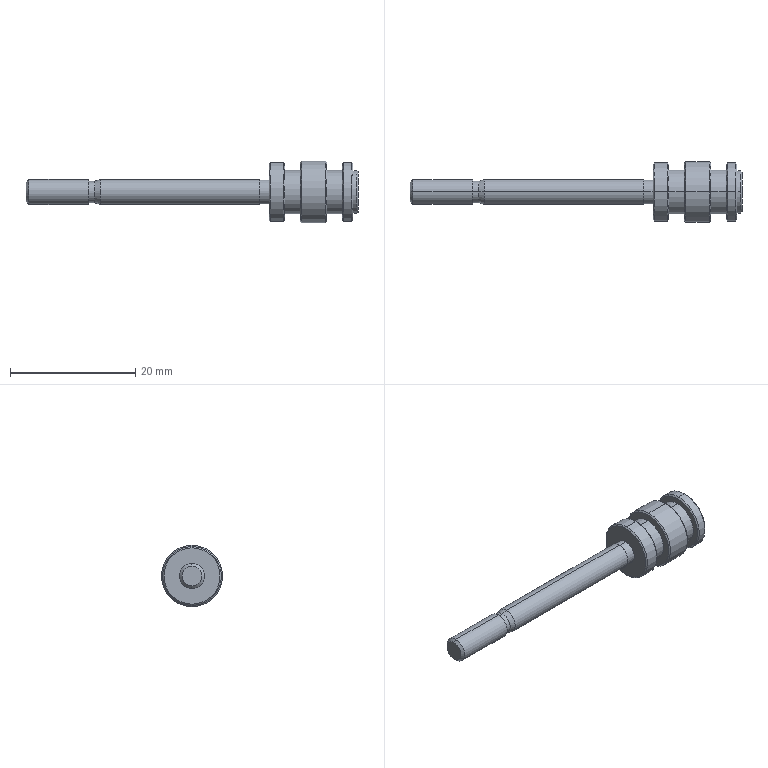Component | SolidWorks | MD-10x10-S-G1-2 (0)-1_MD 10x10-S10 - Rod-1 | 1 solid | 48 faces | box 53 x 9.8 x 9.8 mm | volume 1305 mm3 | cylinder 20 | cone 18 | plane 10 | commonest cylinder face diameters 9.4 x4 7 x4 4 x4 6.8 x2 9.8 x2 3.8 x2 3.4 x2
build123d program:
from build123d import *


with BuildPart() as part:
    # Sketch1 → Revolve1 (revolve)
    with BuildSketch(Plane.XY, mode=Mode.PRIVATE) as revolve1_sk:
        Polygon((-16, 0), (-16, 1.571), (-15.57, 2), (-6, 2), (-6, 1.7), (-5, 1.7), (-4.176, 2), (21.3, 2), (21.3, 1.9), (22.8, 1.9), (22.8, 4.5), (23, 4.7), (25.1, 4.7), (25.3, 4.5), (25.3, 3.5), (27.8, 3.5), (27.8, 4.7), (28, 4.9), (31.8, 4.9), (32, 4.7), (32, 3.5), (34.5, 3.5), (34.5, 4.5), (34.7, 4.7), (36, 4.7), (36.2, 4.5), (36.2, 3.4), (36.8, 3.4), (37, 3.2), (37, 0), align=None)
    revolve(revolve1_sk.sketch.rotate(Axis((37, 0, 0), (-1, 0, 0)), 270), axis=Axis((37, 0, 0), (-1, 0, 0)))


solid = part.part

# Placed as in the assembly
solid = solid.moved(Location((-68.981, 97.516, 82), (0, 0, 0)))